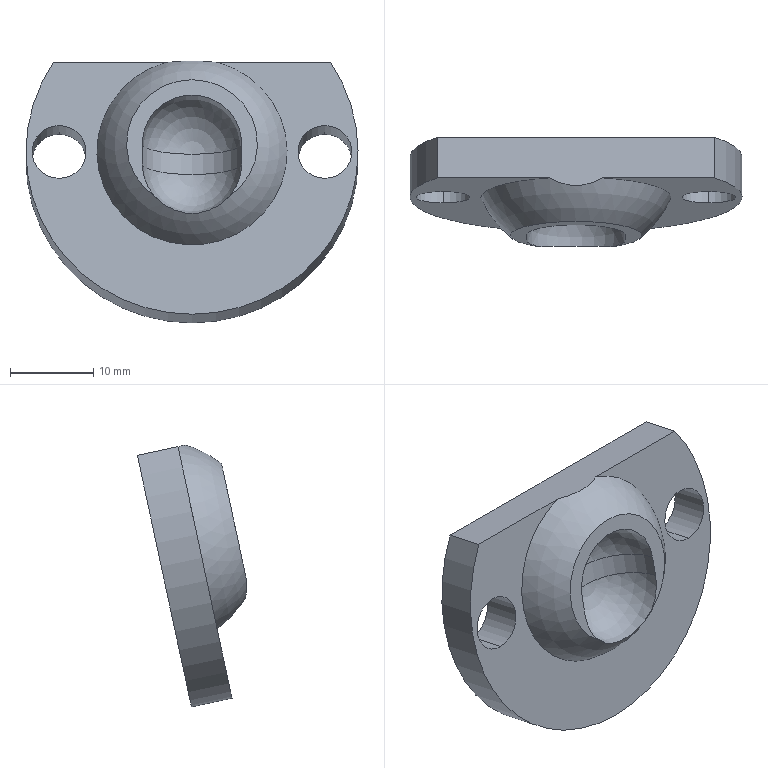Component | SolidWorks | Gland-1 | 1 solid | 13 faces | box 40 x 13.16 x 31.56 mm | volume 5782 mm3 | cylinder 6 | plane 4 | sphere 3 | commonest cylinder face diameters 6.5 x4 40 x1 12 x1
STEP:
#1=CARTESIAN_POINT('',(5.012,2.864,19.491));
#2=VERTEX_POINT('',#1);
#3=CARTESIAN_POINT('',(5.012,2.811,19.241));
#4=VERTEX_POINT('',#3);
#5=CARTESIAN_POINT('',(5.012,2.837,19.366));
#6=DIRECTION('',(-0.,0.9777,-0.2101));
#7=DIRECTION('',(0.,0.2101,0.9777));
#8=AXIS2_PLACEMENT_3D('',#5,#6,#7);
#9=CIRCLE('',#8,0.128);
#10=EDGE_CURVE('',#2,#4,#9,.T.);
#11=ORIENTED_EDGE('',*,*,#10,.T.);
#12=CARTESIAN_POINT('',(5.012,2.618,19.282));
#13=VERTEX_POINT('',#12);
#14=CARTESIAN_POINT('',(5.012,2.811,19.241));
#15=DIRECTION('',(0.,-0.9777,0.2101));
#16=VECTOR('',#15,39.37);
#17=LINE('',#14,#16);
#18=EDGE_CURVE('',#4,#13,#17,.T.);
#19=ORIENTED_EDGE('',*,*,#18,.T.);
#20=CARTESIAN_POINT('',(5.012,2.672,19.532));
#21=VERTEX_POINT('',#20);
#22=CARTESIAN_POINT('',(5.012,2.645,19.407));
#23=DIRECTION('',(-0.,0.9777,-0.2101));
#24=DIRECTION('',(0.,0.2101,0.9777));
#25=AXIS2_PLACEMENT_3D('',#22,#23,#24);
#26=CIRCLE('',#25,0.128);
#27=EDGE_CURVE('',#21,#13,#26,.T.);
#28=ORIENTED_EDGE('',*,*,#27,.F.);
#29=CARTESIAN_POINT('',(5.012,2.864,19.491));
#30=DIRECTION('',(0.,-0.9777,0.2101));
#31=VECTOR('',#30,39.37);
#32=LINE('',#29,#31);
#33=EDGE_CURVE('',#2,#21,#32,.T.);
#34=ORIENTED_EDGE('',*,*,#33,.F.);
#35=EDGE_LOOP('',(#11,#19,#28,#34));
#36=FACE_OUTER_BOUND('',#35,.T.);
#37=CARTESIAN_POINT('',(5.012,2.837,19.366));
#38=DIRECTION('',(0.,-0.9777,0.2101));
#39=DIRECTION('',(0.,0.2101,0.9777));
#40=AXIS2_PLACEMENT_3D('',#37,#38,#39);
#41=CYLINDRICAL_SURFACE('',#40,0.128);
#42=ADVANCED_FACE('',(#36),#41,.F.);
#43=CARTESIAN_POINT('',(3.752,2.864,19.491));
#44=VERTEX_POINT('',#43);
#45=CARTESIAN_POINT('',(3.752,2.811,19.241));
#46=VERTEX_POINT('',#45);
#47=CARTESIAN_POINT('',(3.752,2.837,19.366));
#48=DIRECTION('',(-0.,0.9777,-0.2101));
#49=DIRECTION('',(-0.,-0.2101,-0.9777));
#50=AXIS2_PLACEMENT_3D('',#47,#48,#49);
#51=CIRCLE('',#50,0.128);
#52=EDGE_CURVE('',#44,#46,#51,.T.);
#53=ORIENTED_EDGE('',*,*,#52,.T.);
#54=CARTESIAN_POINT('',(3.752,2.618,19.282));
#55=VERTEX_POINT('',#54);
#56=CARTESIAN_POINT('',(3.752,2.811,19.241));
#57=DIRECTION('',(0.,-0.9777,0.2101));
#58=VECTOR('',#57,39.37);
#59=LINE('',#56,#58);
#60=EDGE_CURVE('',#46,#55,#59,.T.);
#61=ORIENTED_EDGE('',*,*,#60,.T.);
#62=CARTESIAN_POINT('',(3.752,2.672,19.532));
#63=VERTEX_POINT('',#62);
#64=CARTESIAN_POINT('',(3.752,2.645,19.407));
#65=DIRECTION('',(-0.,0.9777,-0.2101));
#66=DIRECTION('',(-0.,-0.2101,-0.9777));
#67=AXIS2_PLACEMENT_3D('',#64,#65,#66);
#68=CIRCLE('',#67,0.128);
#69=EDGE_CURVE('',#63,#55,#68,.T.);
#70=ORIENTED_EDGE('',*,*,#69,.F.);
#71=CARTESIAN_POINT('',(3.752,2.864,19.491));
#72=DIRECTION('',(0.,-0.9777,0.2101));
#73=VECTOR('',#72,39.37);
#74=LINE('',#71,#73);
#75=EDGE_CURVE('',#44,#63,#74,.T.);
#76=ORIENTED_EDGE('',*,*,#75,.F.);
#77=EDGE_LOOP('',(#53,#61,#70,#76));
#78=FACE_OUTER_BOUND('',#77,.T.);
#79=CARTESIAN_POINT('',(3.752,2.837,19.366));
#80=DIRECTION('',(0.,-0.9777,0.2101));
#81=DIRECTION('',(0.,0.2101,0.9777));
#82=AXIS2_PLACEMENT_3D('',#79,#80,#81);
#83=CYLINDRICAL_SURFACE('',#82,0.128);
#84=ADVANCED_FACE('',(#78),#83,.F.);
#85=ORIENTED_EDGE('',*,*,#10,.F.);
#86=CARTESIAN_POINT('',(5.012,2.837,19.366));
#87=DIRECTION('',(-0.,0.9777,-0.2101));
#88=DIRECTION('',(0.,0.2101,0.9777));
#89=AXIS2_PLACEMENT_3D('',#86,#87,#88);
#90=CIRCLE('',#89,0.128);
#91=EDGE_CURVE('',#4,#2,#90,.T.);
#92=ORIENTED_EDGE('',*,*,#91,.F.);
#93=EDGE_LOOP('',(#85,#92));
#94=FACE_BOUND('',#93,.T.);
#95=ORIENTED_EDGE('',*,*,#52,.F.);
#96=CARTESIAN_POINT('',(3.752,2.837,19.366));
#97=DIRECTION('',(-0.,0.9777,-0.2101));
#98=DIRECTION('',(-0.,-0.2101,-0.9777));
#99=AXIS2_PLACEMENT_3D('',#96,#97,#98);
#100=CIRCLE('',#99,0.128);
#101=EDGE_CURVE('',#46,#44,#100,.T.);
#102=ORIENTED_EDGE('',*,*,#101,.F.);
#103=EDGE_LOOP('',(#95,#102));
#104=FACE_BOUND('',#103,.T.);
#105=CARTESIAN_POINT('',(5.039,2.928,19.789));
#106=VERTEX_POINT('',#105);
#107=CARTESIAN_POINT('',(3.724,2.928,19.789));
#108=VERTEX_POINT('',#107);
#109=CARTESIAN_POINT('',(4.382,2.837,19.366));
#110=DIRECTION('',(-0.,0.9777,-0.2101));
#111=DIRECTION('',(-0.,-0.2101,-0.9777));
#112=AXIS2_PLACEMENT_3D('',#109,#110,#111);
#113=CIRCLE('',#112,0.7874);
#114=EDGE_CURVE('',#106,#108,#113,.T.);
#115=ORIENTED_EDGE('',*,*,#114,.T.);
#116=CARTESIAN_POINT('',(3.724,2.928,19.789));
#117=DIRECTION('',(-1.,-0.,0.));
#118=VECTOR('',#117,39.37);
#119=LINE('',#116,#118);
#120=EDGE_CURVE('',#106,#108,#119,.T.);
#121=ORIENTED_EDGE('',*,*,#120,.F.);
#122=EDGE_LOOP('',(#115,#121));
#123=FACE_OUTER_BOUND('',#122,.T.);
#124=CARTESIAN_POINT('',(4.382,2.837,19.366));
#125=DIRECTION('',(-0.,0.9777,-0.2101));
#126=DIRECTION('',(-0.,-0.2101,-0.9777));
#127=AXIS2_PLACEMENT_3D('',#124,#125,#126);
#128=PLANE('',#127);
#129=ADVANCED_FACE('',(#94,#104,#123),#128,.T.);
#130=ORIENTED_EDGE('',*,*,#120,.T.);
#131=CARTESIAN_POINT('',(3.724,2.736,19.831));
#132=VERTEX_POINT('',#131);
#133=CARTESIAN_POINT('',(3.724,2.736,19.831));
#134=DIRECTION('',(-0.,0.9777,-0.2101));
#135=VECTOR('',#134,39.37);
#136=LINE('',#133,#135);
#137=EDGE_CURVE('',#132,#108,#136,.T.);
#138=ORIENTED_EDGE('',*,*,#137,.F.);
#139=CARTESIAN_POINT('',(4.256,2.736,19.831));
#140=VERTEX_POINT('',#139);
#141=CARTESIAN_POINT('',(3.724,2.736,19.831));
#142=DIRECTION('',(1.,0.,-0.));
#143=VECTOR('',#142,39.37);
#144=LINE('',#141,#143);
#145=EDGE_CURVE('',#132,#140,#144,.T.);
#146=ORIENTED_EDGE('',*,*,#145,.T.);
#147=CARTESIAN_POINT('',(4.508,2.736,19.831));
#148=VERTEX_POINT('',#147);
#149=CARTESIAN_POINT('',(4.382,2.928,19.789));
#150=DIRECTION('',(-0.,-0.2101,-0.9777));
#151=DIRECTION('',(-1.,0.,0.));
#152=AXIS2_PLACEMENT_3D('',#149,#150,#151);
#153=CIRCLE('',#152,0.2337);
#154=EDGE_CURVE('',#148,#140,#153,.T.);
#155=ORIENTED_EDGE('',*,*,#154,.F.);
#156=CARTESIAN_POINT('',(5.039,2.736,19.831));
#157=VERTEX_POINT('',#156);
#158=CARTESIAN_POINT('',(3.724,2.736,19.831));
#159=DIRECTION('',(1.,0.,-0.));
#160=VECTOR('',#159,39.37);
#161=LINE('',#158,#160);
#162=EDGE_CURVE('',#148,#157,#161,.T.);
#163=ORIENTED_EDGE('',*,*,#162,.T.);
#164=CARTESIAN_POINT('',(5.039,2.736,19.831));
#165=DIRECTION('',(-0.,0.9777,-0.2101));
#166=VECTOR('',#165,39.37);
#167=LINE('',#164,#166);
#168=EDGE_CURVE('',#157,#106,#167,.T.);
#169=ORIENTED_EDGE('',*,*,#168,.T.);
#170=EDGE_LOOP('',(#130,#138,#146,#155,#163,#169));
#171=FACE_OUTER_BOUND('',#170,.T.);
#172=CARTESIAN_POINT('',(3.724,2.736,19.831));
#173=DIRECTION('',(-0.,-0.2101,-0.9777));
#174=DIRECTION('',(-1.,-0.,0.));
#175=AXIS2_PLACEMENT_3D('',#172,#173,#174);
#176=PLANE('',#175);
#177=ADVANCED_FACE('',(#171),#176,.F.);
#178=CARTESIAN_POINT('',(4.382,2.645,19.407));
#179=DIRECTION('',(0.,-0.9777,0.2101));
#180=DIRECTION('',(-0.,-0.2101,-0.9777));
#181=AXIS2_PLACEMENT_3D('',#178,#179,#180);
#182=CIRCLE('',#181,0.451);
#183=EDGE_CURVE('',#140,#148,#182,.T.);
#184=ORIENTED_EDGE('',*,*,#183,.F.);
#185=ORIENTED_EDGE('',*,*,#145,.F.);
#186=CARTESIAN_POINT('',(4.382,2.645,19.407));
#187=DIRECTION('',(-0.,0.9777,-0.2101));
#188=DIRECTION('',(-0.,-0.2101,-0.9777));
#189=AXIS2_PLACEMENT_3D('',#186,#187,#188);
#190=CIRCLE('',#189,0.7874);
#191=EDGE_CURVE('',#157,#132,#190,.T.);
#192=ORIENTED_EDGE('',*,*,#191,.F.);
#193=ORIENTED_EDGE('',*,*,#162,.F.);
#194=EDGE_LOOP('',(#184,#185,#192,#193));
#195=FACE_OUTER_BOUND('',#194,.T.);
#196=ORIENTED_EDGE('',*,*,#69,.T.);
#197=CARTESIAN_POINT('',(3.752,2.645,19.407));
#198=DIRECTION('',(-0.,0.9777,-0.2101));
#199=DIRECTION('',(-0.,-0.2101,-0.9777));
#200=AXIS2_PLACEMENT_3D('',#197,#198,#199);
#201=CIRCLE('',#200,0.128);
#202=EDGE_CURVE('',#55,#63,#201,.T.);
#203=ORIENTED_EDGE('',*,*,#202,.T.);
#204=EDGE_LOOP('',(#196,#203));
#205=FACE_BOUND('',#204,.T.);
#206=ORIENTED_EDGE('',*,*,#27,.T.);
#207=CARTESIAN_POINT('',(5.012,2.645,19.407));
#208=DIRECTION('',(-0.,0.9777,-0.2101));
#209=DIRECTION('',(0.,0.2101,0.9777));
#210=AXIS2_PLACEMENT_3D('',#207,#208,#209);
#211=CIRCLE('',#210,0.128);
#212=EDGE_CURVE('',#13,#21,#211,.T.);
#213=ORIENTED_EDGE('',*,*,#212,.T.);
#214=EDGE_LOOP('',(#206,#213));
#215=FACE_BOUND('',#214,.T.);
#216=CARTESIAN_POINT('',(4.382,2.645,19.407));
#217=DIRECTION('',(-0.,0.9777,-0.2101));
#218=DIRECTION('',(-0.,-0.2101,-0.9777));
#219=AXIS2_PLACEMENT_3D('',#216,#217,#218);
#220=PLANE('',#219);
#221=ADVANCED_FACE('',(#195,#205,#215),#220,.F.);
#222=ORIENTED_EDGE('',*,*,#114,.F.);
#223=ORIENTED_EDGE('',*,*,#168,.F.);
#224=ORIENTED_EDGE('',*,*,#191,.T.);
#225=ORIENTED_EDGE('',*,*,#137,.T.);
#226=EDGE_LOOP('',(#222,#223,#224,#225));
#227=FACE_OUTER_BOUND('',#226,.T.);
#228=CARTESIAN_POINT('',(4.382,2.837,19.366));
#229=DIRECTION('',(0.,-0.9777,0.2101));
#230=DIRECTION('',(0.,0.2101,0.9777));
#231=AXIS2_PLACEMENT_3D('',#228,#229,#230);
#232=CYLINDRICAL_SURFACE('',#231,0.7874);
#233=ADVANCED_FACE('',(#227),#232,.T.);
#234=ORIENTED_EDGE('',*,*,#60,.F.);
#235=ORIENTED_EDGE('',*,*,#101,.T.);
#236=ORIENTED_EDGE('',*,*,#75,.T.);
#237=ORIENTED_EDGE('',*,*,#202,.F.);
#238=EDGE_LOOP('',(#234,#235,#236,#237));
#239=FACE_OUTER_BOUND('',#238,.T.);
#240=CARTESIAN_POINT('',(3.752,2.837,19.366));
#241=DIRECTION('',(0.,-0.9777,0.2101));
#242=DIRECTION('',(0.,0.2101,0.9777));
#243=AXIS2_PLACEMENT_3D('',#240,#241,#242);
#244=CYLINDRICAL_SURFACE('',#243,0.128);
#245=ADVANCED_FACE('',(#239),#244,.F.);
#246=ORIENTED_EDGE('',*,*,#18,.F.);
#247=ORIENTED_EDGE('',*,*,#91,.T.);
#248=ORIENTED_EDGE('',*,*,#33,.T.);
#249=ORIENTED_EDGE('',*,*,#212,.F.);
#250=EDGE_LOOP('',(#246,#247,#248,#249));
#251=FACE_OUTER_BOUND('',#250,.T.);
#252=CARTESIAN_POINT('',(5.012,2.837,19.366));
#253=DIRECTION('',(0.,-0.9777,0.2101));
#254=DIRECTION('',(0.,0.2101,0.9777));
#255=AXIS2_PLACEMENT_3D('',#252,#253,#254);
#256=CYLINDRICAL_SURFACE('',#255,0.128);
#257=ADVANCED_FACE('',(#251),#256,.F.);
#258=CARTESIAN_POINT('',(4.205,2.41,19.197));
#259=VERTEX_POINT('',#258);
#260=CARTESIAN_POINT('',(4.558,2.41,19.197));
#261=VERTEX_POINT('',#260);
#262=CARTESIAN_POINT('',(4.382,2.464,19.446));
#263=DIRECTION('',(-0.,0.9777,-0.2101));
#264=DIRECTION('',(1.,0.,-0.));
#265=AXIS2_PLACEMENT_3D('',#262,#263,#264);
#266=CIRCLE('',#265,0.3104);
#267=EDGE_CURVE('',#259,#261,#266,.T.);
#268=ORIENTED_EDGE('',*,*,#267,.T.);
#269=CARTESIAN_POINT('',(4.382,2.404,19.348));
#270=DIRECTION('',(0.,0.9992,0.04057));
#271=DIRECTION('',(0.,-0.04057,0.9992));
#272=AXIS2_PLACEMENT_3D('',#269,#270,#271);
#273=CIRCLE('',#272,0.233);
#274=EDGE_CURVE('',#261,#259,#273,.T.);
#275=ORIENTED_EDGE('',*,*,#274,.T.);
#276=EDGE_LOOP('',(#268,#275));
#277=FACE_BOUND('',#276,.T.);
#278=ORIENTED_EDGE('',*,*,#183,.T.);
#279=ORIENTED_EDGE('',*,*,#154,.T.);
#280=EDGE_LOOP('',(#278,#279));
#281=FACE_OUTER_BOUND('',#280,.T.);
#282=CARTESIAN_POINT('',(4.382,2.837,19.366));
#283=DIRECTION('',(0.,-0.9777,0.2101));
#284=DIRECTION('',(-0.,-0.2101,-0.9777));
#285=AXIS2_PLACEMENT_3D('',#282,#283,#284);
#286=SPHERICAL_SURFACE('',#285,0.4921);
#287=ADVANCED_FACE('',(#277,#281),#286,.T.);
#288=CARTESIAN_POINT('',(4.618,2.464,19.446));
#289=VERTEX_POINT('',#288);
#290=CARTESIAN_POINT('',(4.618,2.443,19.35));
#291=VERTEX_POINT('',#290);
#292=CARTESIAN_POINT('',(4.618,2.464,19.446));
#293=DIRECTION('',(-0.,-0.2101,-0.9777));
#294=VECTOR('',#293,39.37);
#295=LINE('',#292,#294);
#296=EDGE_CURVE('',#289,#291,#295,.T.);
#297=ORIENTED_EDGE('',*,*,#296,.T.);
#298=CARTESIAN_POINT('',(4.382,2.443,19.35));
#299=DIRECTION('',(-0.,0.9777,-0.2101));
#300=DIRECTION('',(1.,0.,-0.));
#301=AXIS2_PLACEMENT_3D('',#298,#299,#300);
#302=CIRCLE('',#301,0.2362);
#303=EDGE_CURVE('',#291,#261,#302,.T.);
#304=ORIENTED_EDGE('',*,*,#303,.T.);
#305=ORIENTED_EDGE('',*,*,#267,.F.);
#306=CARTESIAN_POINT('',(4.146,2.443,19.35));
#307=VERTEX_POINT('',#306);
#308=CARTESIAN_POINT('',(4.382,2.443,19.35));
#309=DIRECTION('',(-0.,0.9777,-0.2101));
#310=DIRECTION('',(1.,0.,-0.));
#311=AXIS2_PLACEMENT_3D('',#308,#309,#310);
#312=CIRCLE('',#311,0.2362);
#313=EDGE_CURVE('',#259,#307,#312,.T.);
#314=ORIENTED_EDGE('',*,*,#313,.T.);
#315=CARTESIAN_POINT('',(4.146,2.464,19.446));
#316=VERTEX_POINT('',#315);
#317=CARTESIAN_POINT('',(4.146,2.464,19.446));
#318=DIRECTION('',(0.,0.2101,0.9777));
#319=VECTOR('',#318,39.37);
#320=LINE('',#317,#319);
#321=EDGE_CURVE('',#307,#316,#320,.T.);
#322=ORIENTED_EDGE('',*,*,#321,.T.);
#323=CARTESIAN_POINT('',(4.382,2.464,19.446));
#324=DIRECTION('',(-0.,0.9777,-0.2101));
#325=DIRECTION('',(1.,0.,-0.));
#326=AXIS2_PLACEMENT_3D('',#323,#324,#325);
#327=CIRCLE('',#326,0.2362);
#328=EDGE_CURVE('',#316,#289,#327,.T.);
#329=ORIENTED_EDGE('',*,*,#328,.T.);
#330=EDGE_LOOP('',(#297,#304,#305,#314,#322,#329));
#331=FACE_OUTER_BOUND('',#330,.T.);
#332=CARTESIAN_POINT('',(3.904,2.299,18.676));
#333=DIRECTION('',(-0.,0.9777,-0.2101));
#334=DIRECTION('',(1.,0.,-0.));
#335=AXIS2_PLACEMENT_3D('',#332,#333,#334);
#336=PLANE('',#335);
#337=ADVANCED_FACE('',(#331),#336,.F.);
#338=CARTESIAN_POINT('',(4.382,2.464,19.446));
#339=DIRECTION('',(0.,0.2101,0.9777));
#340=DIRECTION('',(1.,0.,-0.));
#341=AXIS2_PLACEMENT_3D('',#338,#339,#340);
#342=CIRCLE('',#341,0.2362);
#343=EDGE_CURVE('',#289,#316,#342,.T.);
#344=ORIENTED_EDGE('',*,*,#343,.F.);
#345=ORIENTED_EDGE('',*,*,#328,.F.);
#346=EDGE_LOOP('',(#344,#345));
#347=FACE_OUTER_BOUND('',#346,.T.);
#348=CARTESIAN_POINT('',(4.382,2.464,19.446));
#349=DIRECTION('',(-0.,0.9777,-0.2101));
#350=DIRECTION('',(1.,0.,-0.));
#351=AXIS2_PLACEMENT_3D('',#348,#349,#350);
#352=SPHERICAL_SURFACE('',#351,0.2362);
#353=ADVANCED_FACE('',(#347),#352,.F.);
#354=CARTESIAN_POINT('',(4.382,2.443,19.35));
#355=DIRECTION('',(0.,0.2101,0.9777));
#356=DIRECTION('',(1.,0.,-0.));
#357=AXIS2_PLACEMENT_3D('',#354,#355,#356);
#358=CIRCLE('',#357,0.2362);
#359=EDGE_CURVE('',#291,#307,#358,.T.);
#360=ORIENTED_EDGE('',*,*,#359,.F.);
#361=ORIENTED_EDGE('',*,*,#296,.F.);
#362=ORIENTED_EDGE('',*,*,#343,.T.);
#363=ORIENTED_EDGE('',*,*,#321,.F.);
#364=EDGE_LOOP('',(#360,#361,#362,#363));
#365=FACE_OUTER_BOUND('',#364,.T.);
#366=CARTESIAN_POINT('',(4.382,2.464,19.446));
#367=DIRECTION('',(0.,0.2101,0.9777));
#368=DIRECTION('',(1.,0.,-0.));
#369=AXIS2_PLACEMENT_3D('',#366,#367,#368);
#370=CYLINDRICAL_SURFACE('',#369,0.2362);
#371=ADVANCED_FACE('',(#365),#370,.F.);
#372=ORIENTED_EDGE('',*,*,#359,.T.);
#373=ORIENTED_EDGE('',*,*,#313,.F.);
#374=ORIENTED_EDGE('',*,*,#274,.F.);
#375=ORIENTED_EDGE('',*,*,#303,.F.);
#376=EDGE_LOOP('',(#372,#373,#374,#375));
#377=FACE_OUTER_BOUND('',#376,.T.);
#378=CARTESIAN_POINT('',(4.382,2.443,19.35));
#379=DIRECTION('',(0.,-0.9777,0.2101));
#380=DIRECTION('',(-1.,0.,0.));
#381=AXIS2_PLACEMENT_3D('',#378,#379,#380);
#382=SPHERICAL_SURFACE('',#381,0.2362);
#383=ADVANCED_FACE('',(#377),#382,.F.);
#384=CLOSED_SHELL('',(#42,#84,#129,#177,#221,#233,#245,#257,#287,#337,#353,#371,#383));
#385=MANIFOLD_SOLID_BREP('',#384);
#386=CARTESIAN_POINT('',(0.,0.,0.));
#387=DIRECTION('',(0.,0.,1.));
#388=DIRECTION('',(1.,0.,0.));
#389=AXIS2_PLACEMENT_3D('',#386,#387,#388);
#390=(LENGTH_UNIT()NAMED_UNIT(*)SI_UNIT($,.METRE.));
#391=LENGTH_MEASURE_WITH_UNIT(LENGTH_MEASURE(0.0254),#390);
#392=DIMENSIONAL_EXPONENTS(1.,0.,0.,0.,0.,0.,0.);
#393=(CONVERSION_BASED_UNIT('',#391)LENGTH_UNIT()NAMED_UNIT(#392));
#394=UNCERTAINTY_MEASURE_WITH_UNIT(LENGTH_MEASURE(0.00001),#393,'','');
#395=(NAMED_UNIT(*)PLANE_ANGLE_UNIT()SI_UNIT($,.RADIAN.));
#396=(NAMED_UNIT(*)SI_UNIT($,.STERADIAN.)SOLID_ANGLE_UNIT());
#397=(GEOMETRIC_REPRESENTATION_CONTEXT(3)GLOBAL_UNCERTAINTY_ASSIGNED_CONTEXT((#394))GLOBAL_UNIT_ASSIGNED_CONTEXT((#393,#395,#396))REPRESENTATION_CONTEXT('',''));
#398=ADVANCED_BREP_SHAPE_REPRESENTATION('',(#385,#389),#397);
#399=COLOUR_RGB('',0.7922,0.8196,0.9333);
#400=FILL_AREA_STYLE_COLOUR('',#399);
#401=FILL_AREA_STYLE('',(#400));
#402=SURFACE_STYLE_FILL_AREA(#401);
#403=SURFACE_SIDE_STYLE('',(#402));
#404=SURFACE_STYLE_USAGE(.BOTH.,#403);
#405=PRESENTATION_STYLE_ASSIGNMENT((#404));
#406=STYLED_ITEM('',(#405),#385);
#407=(LENGTH_UNIT()NAMED_UNIT(*)SI_UNIT($,.METRE.));
#408=LENGTH_MEASURE_WITH_UNIT(LENGTH_MEASURE(0.0254),#407);
#409=DIMENSIONAL_EXPONENTS(1.,0.,0.,0.,0.,0.,0.);
#410=(CONVERSION_BASED_UNIT('',#408)LENGTH_UNIT()NAMED_UNIT(#409));
#411=UNCERTAINTY_MEASURE_WITH_UNIT(LENGTH_MEASURE(0.00001),#410,'','');
#412=(NAMED_UNIT(*)PLANE_ANGLE_UNIT()SI_UNIT($,.RADIAN.));
#413=(NAMED_UNIT(*)SI_UNIT($,.STERADIAN.)SOLID_ANGLE_UNIT());
#414=(GEOMETRIC_REPRESENTATION_CONTEXT(3)GLOBAL_UNCERTAINTY_ASSIGNED_CONTEXT((#411))GLOBAL_UNIT_ASSIGNED_CONTEXT((#410,#412,#413))REPRESENTATION_CONTEXT('',''));
#415=MECHANICAL_DESIGN_GEOMETRIC_PRESENTATION_REPRESENTATION('',(#406),#414);
#416=PRESENTATION_LAYER_ASSIGNMENT('','',(#406));